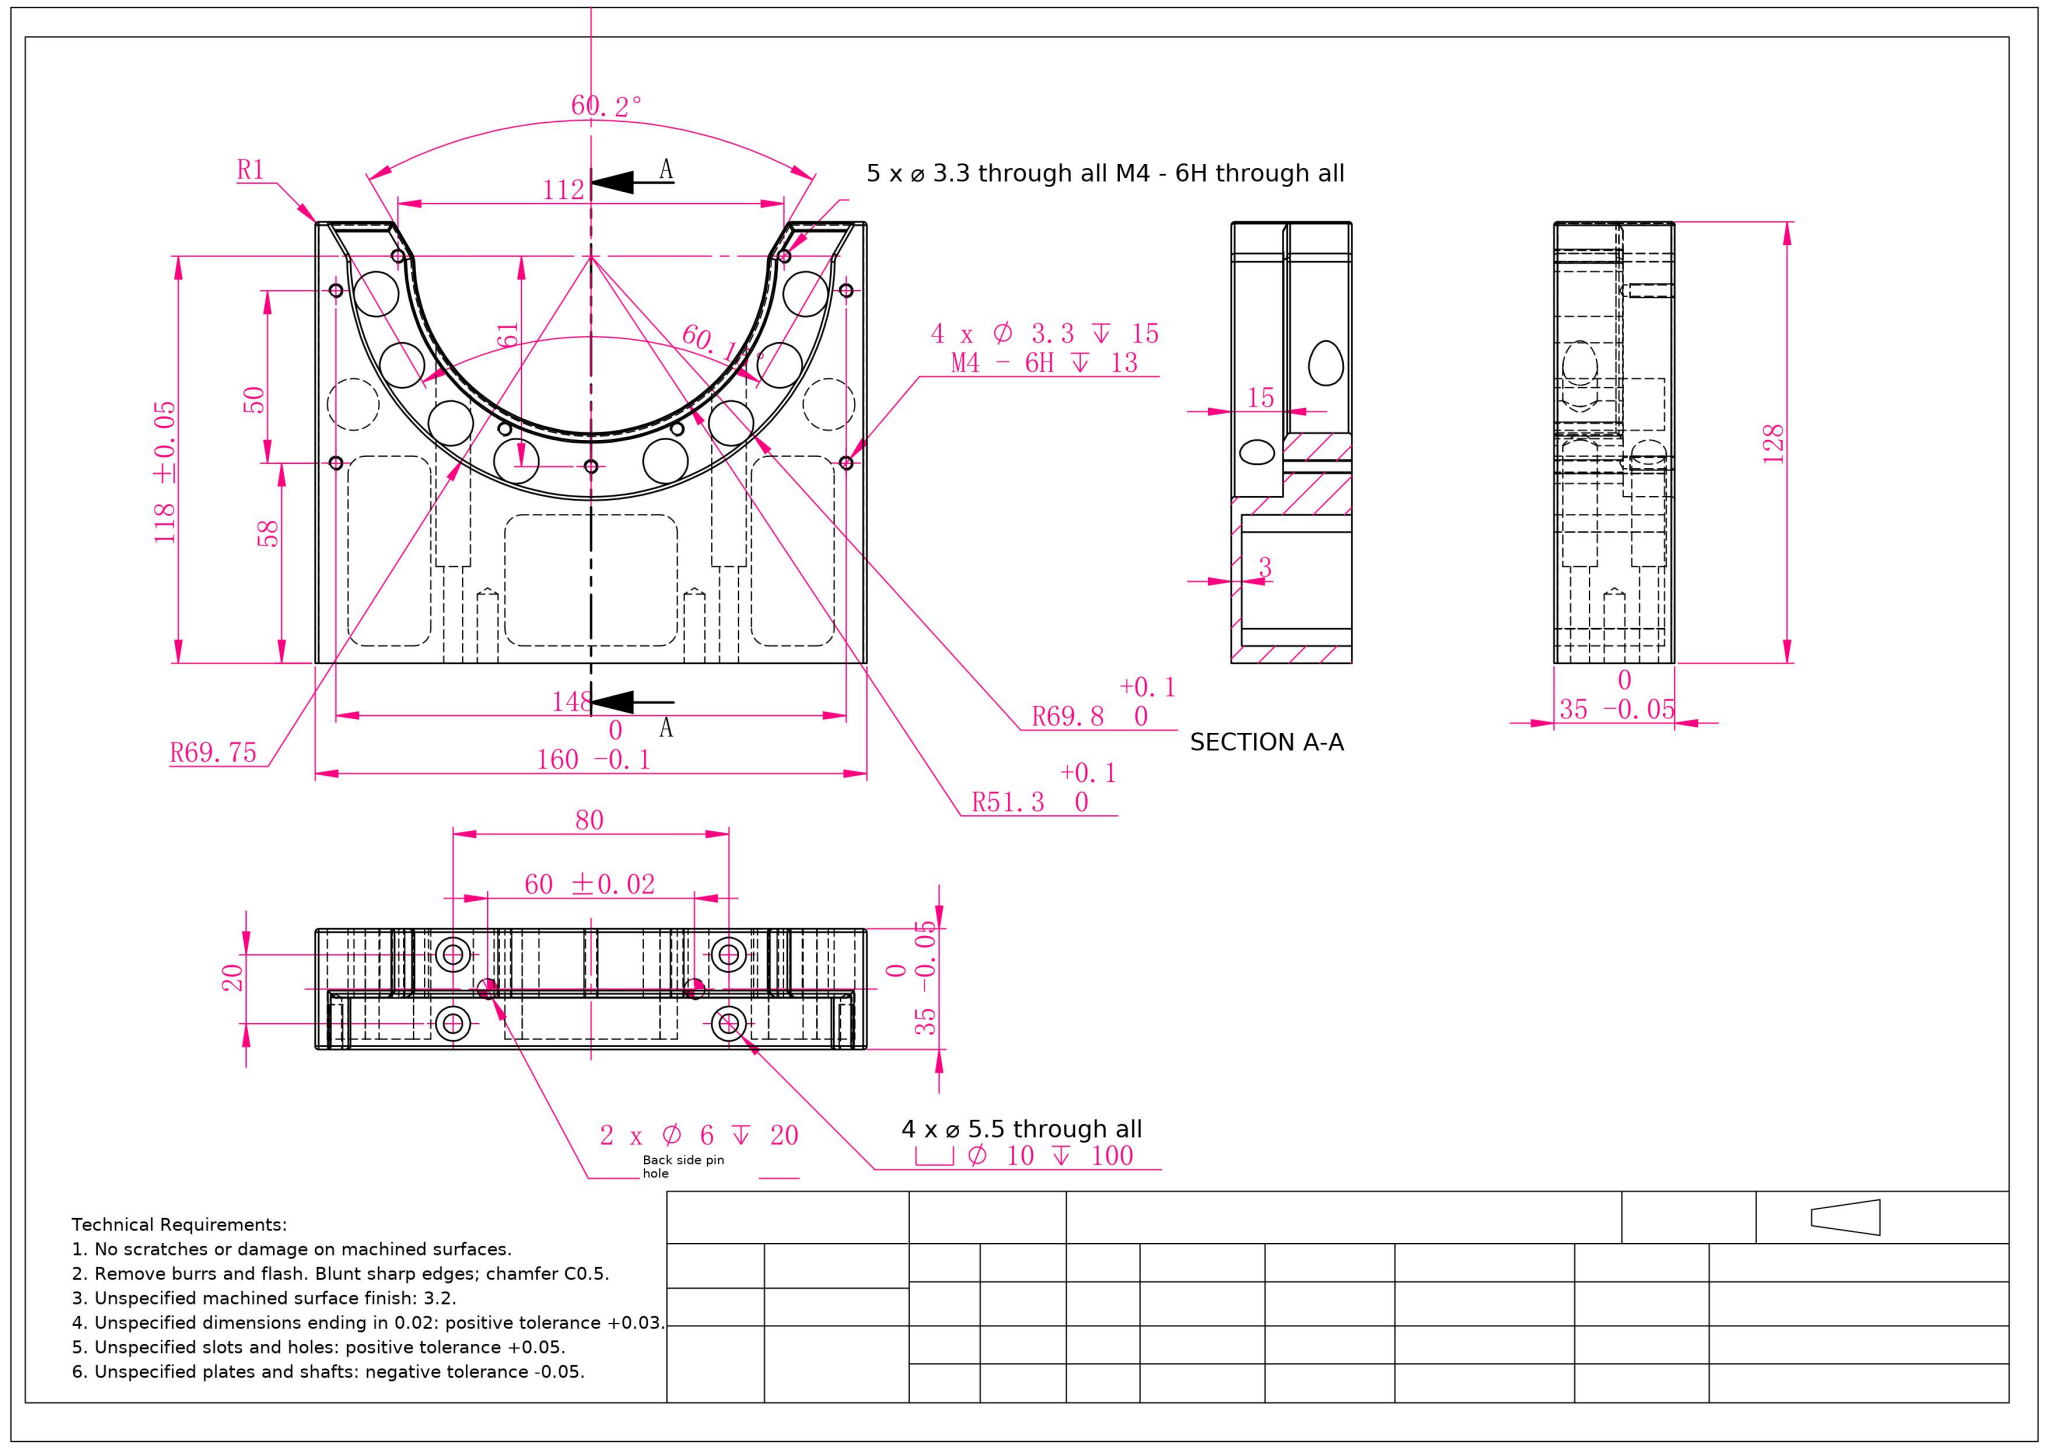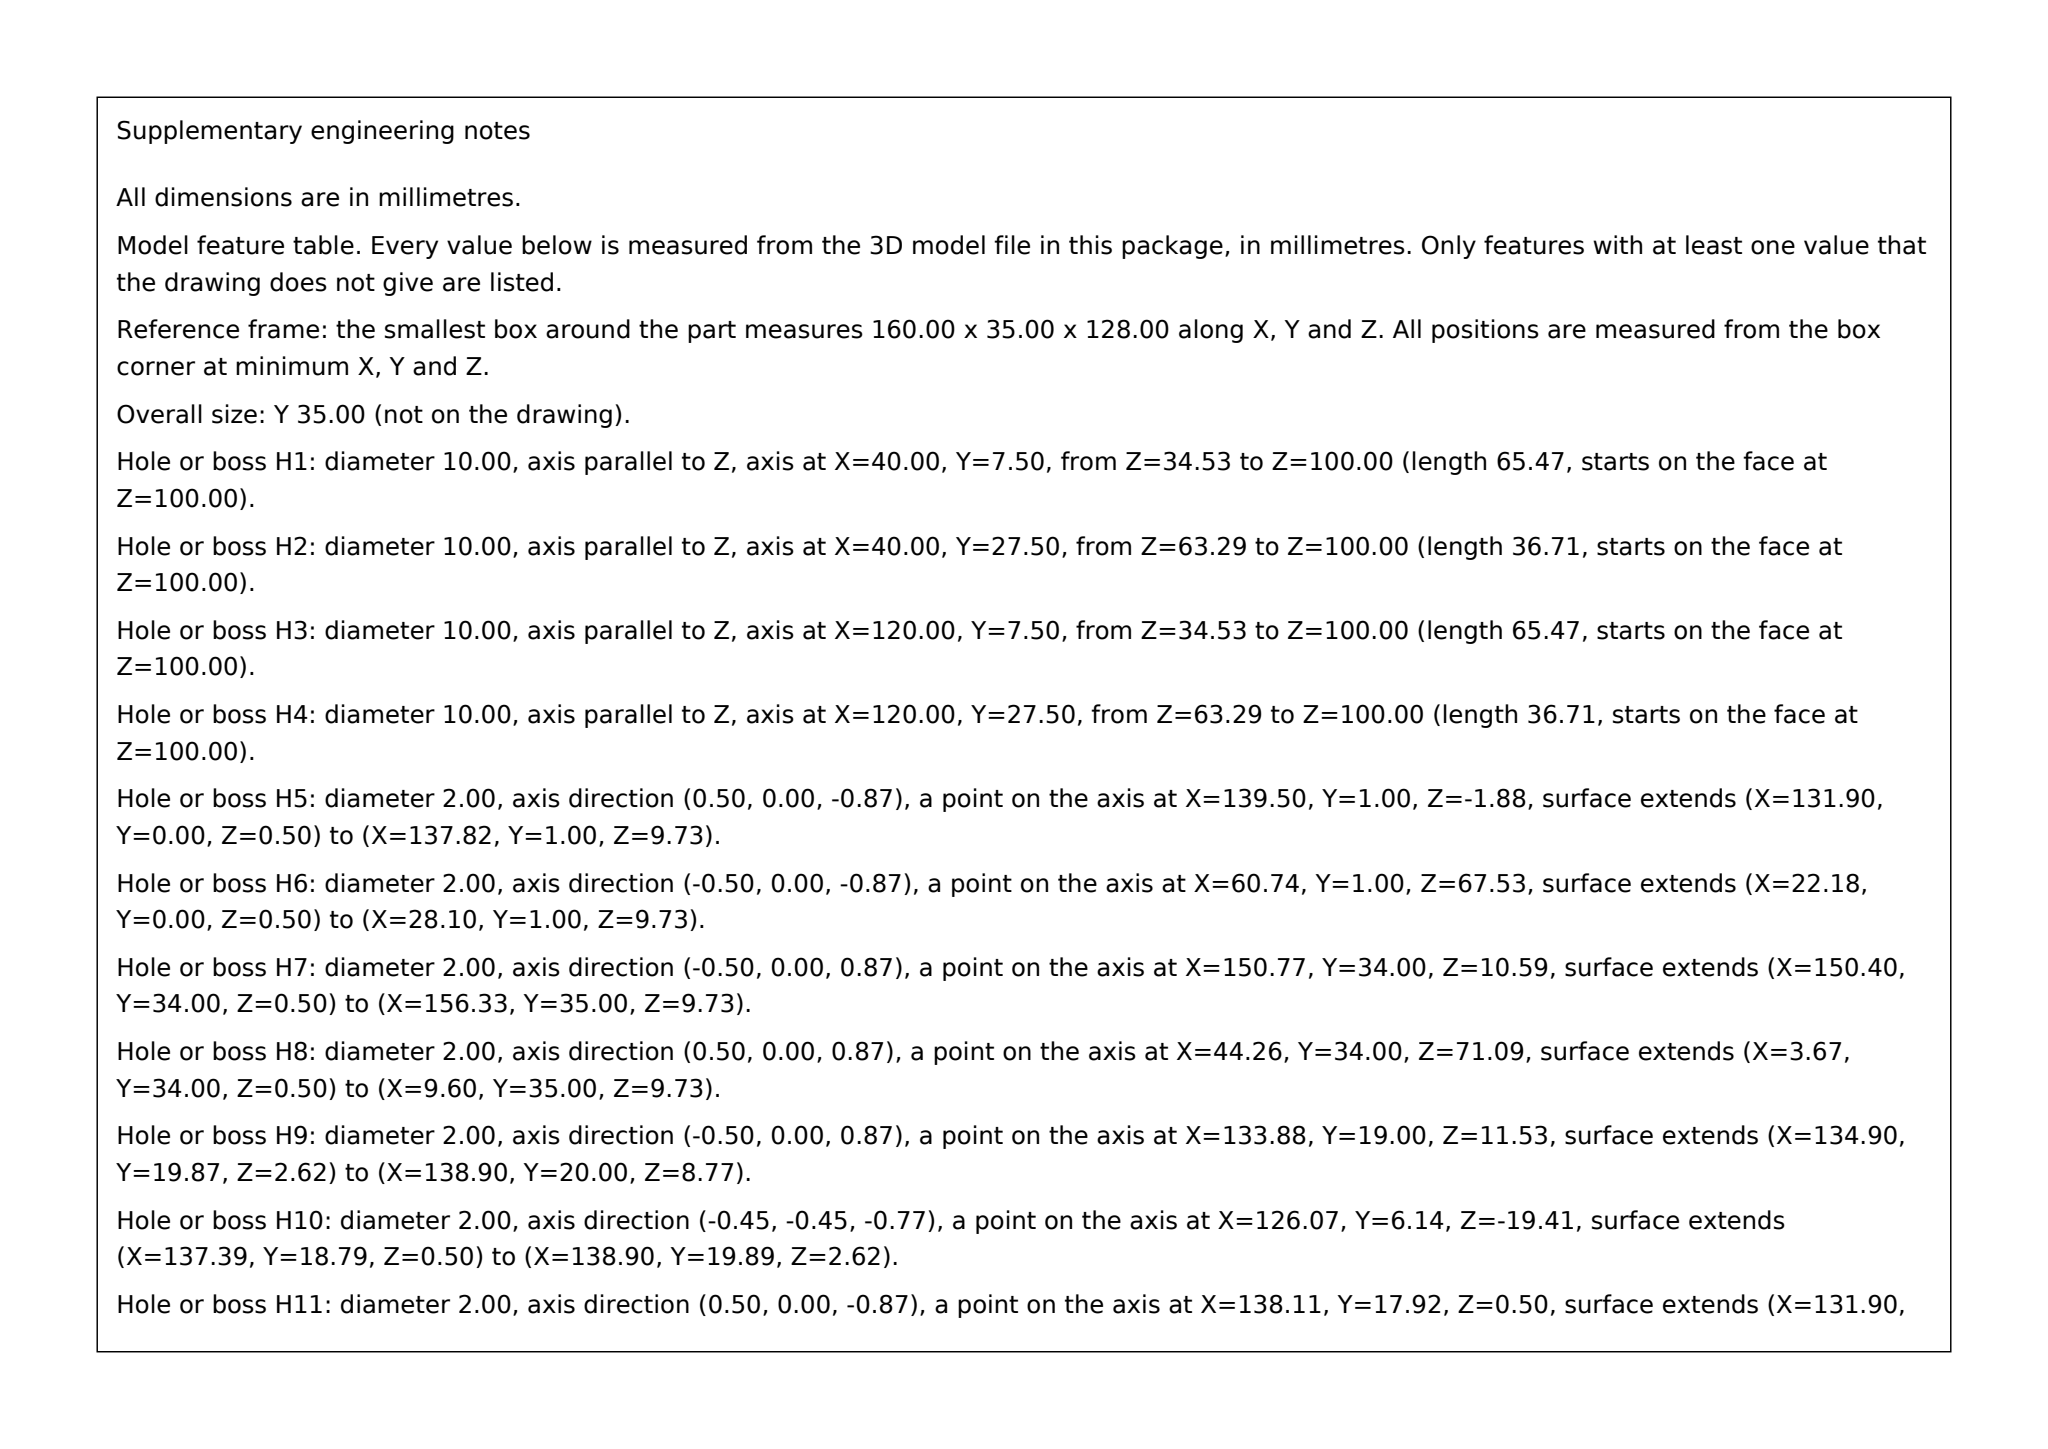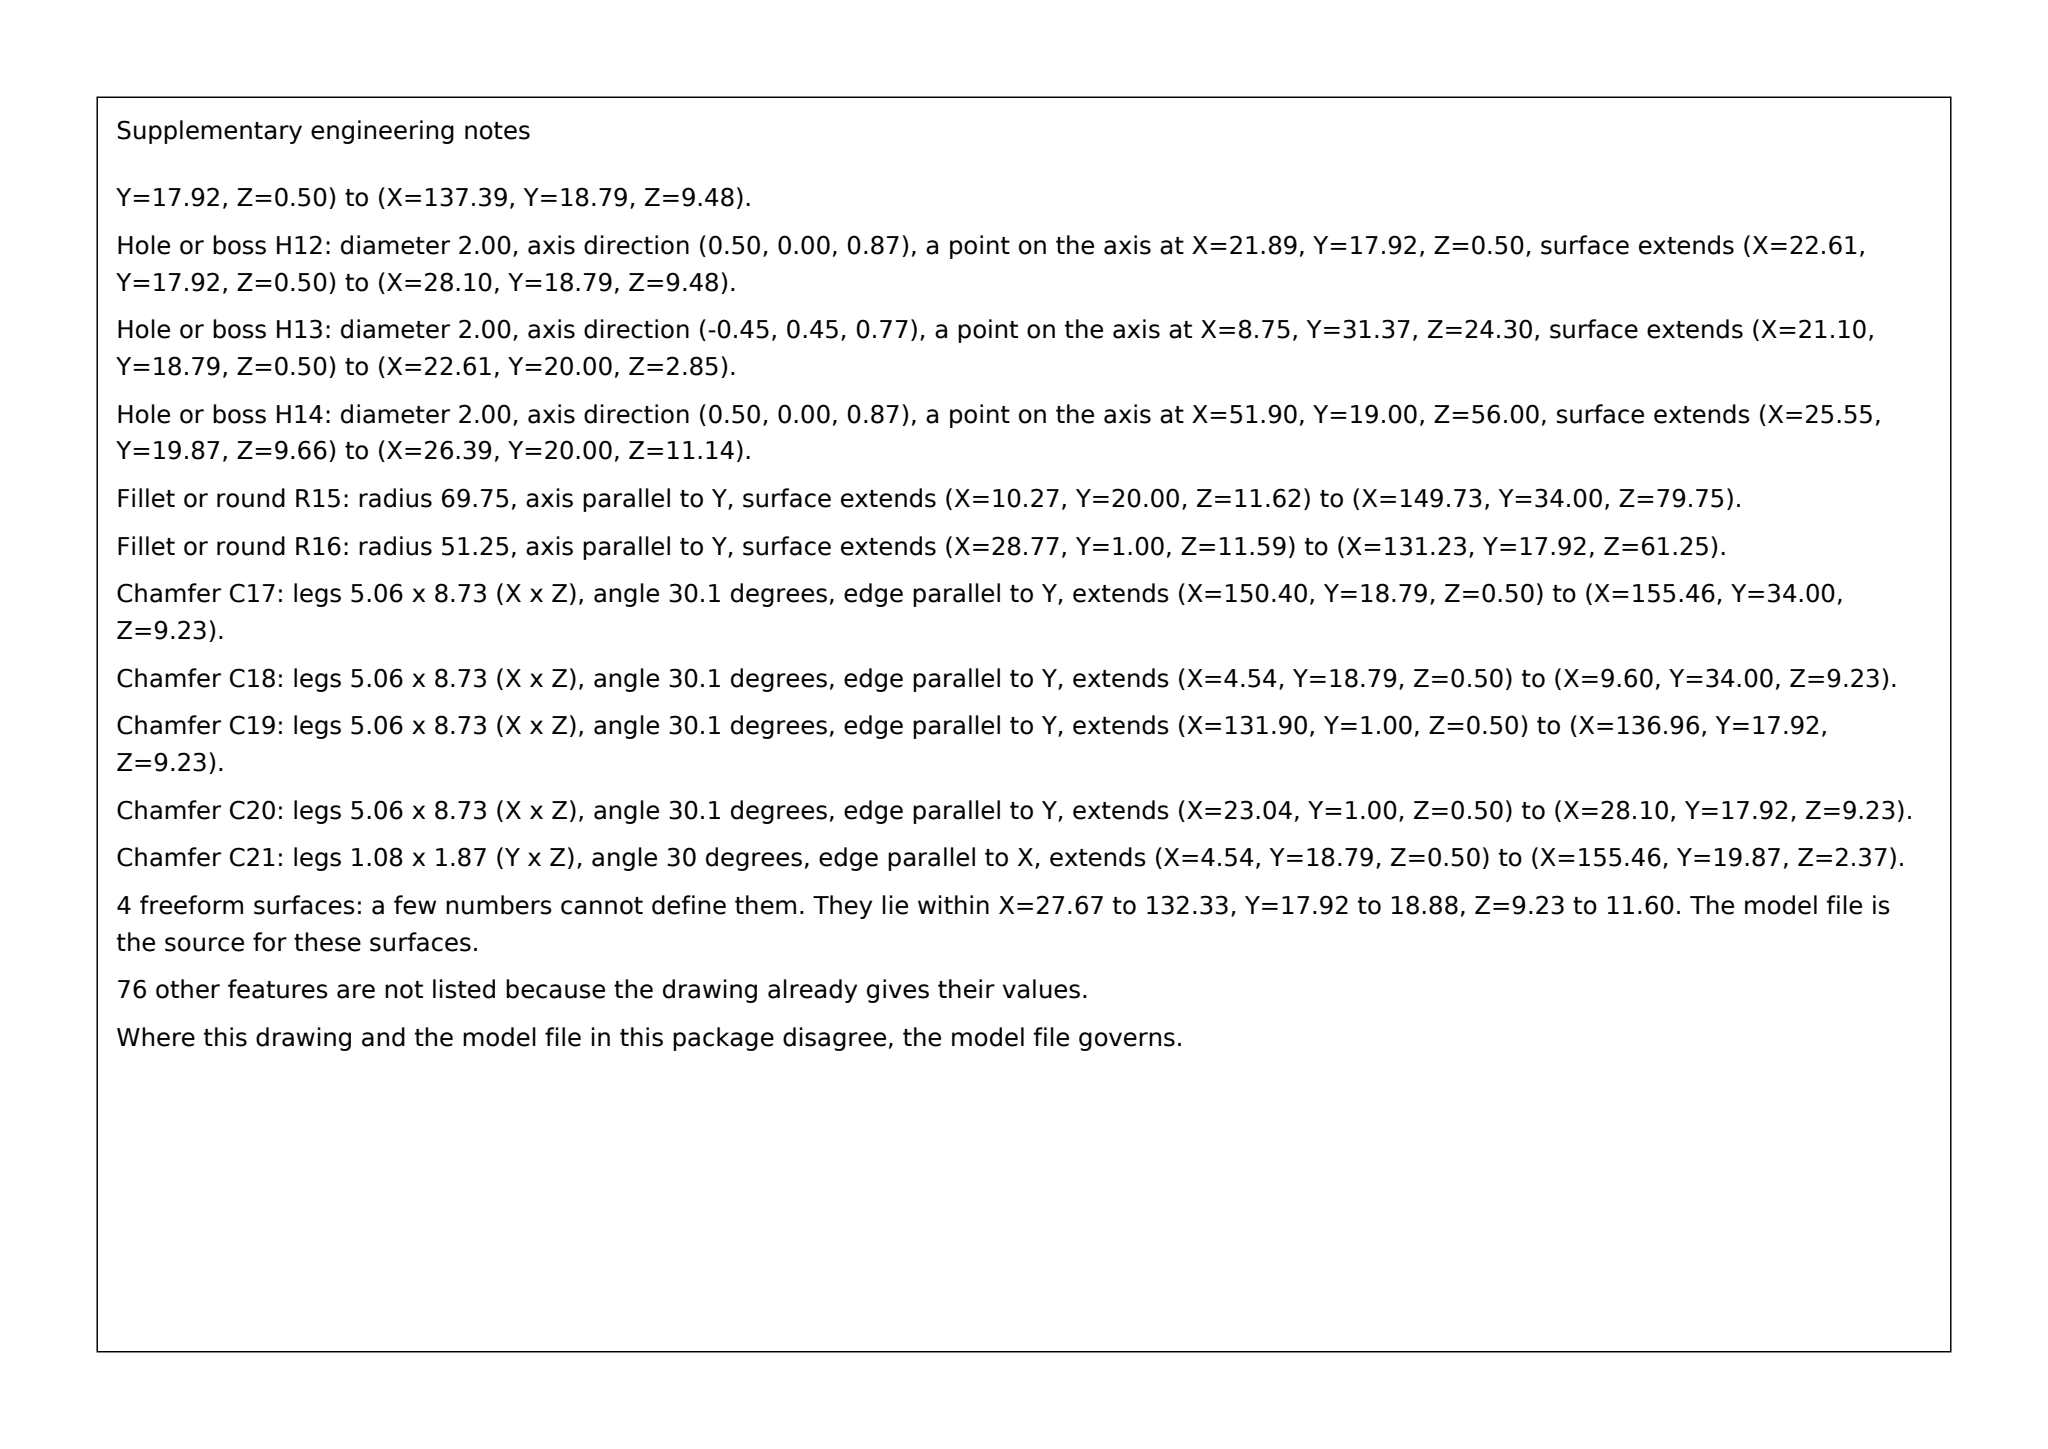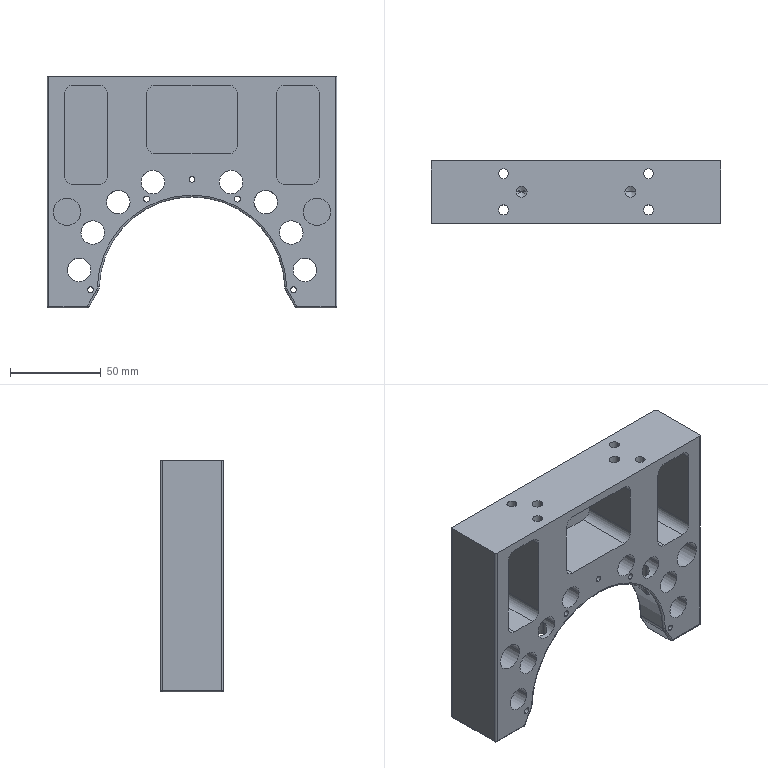Part | SolidWorks | mm | 1 solid | 183 faces | box 160 x 35 x 128 mm | volume 281944 mm3 | cylinder 108 | plane 37 | cone 13 | sphere 13 | torus 8 | spline 4 | commonest cylinder face diameters 10 x28 2 x28 3.3 x18 13 x16 5.5 x8 15 x4 6 x4 102.5 x1